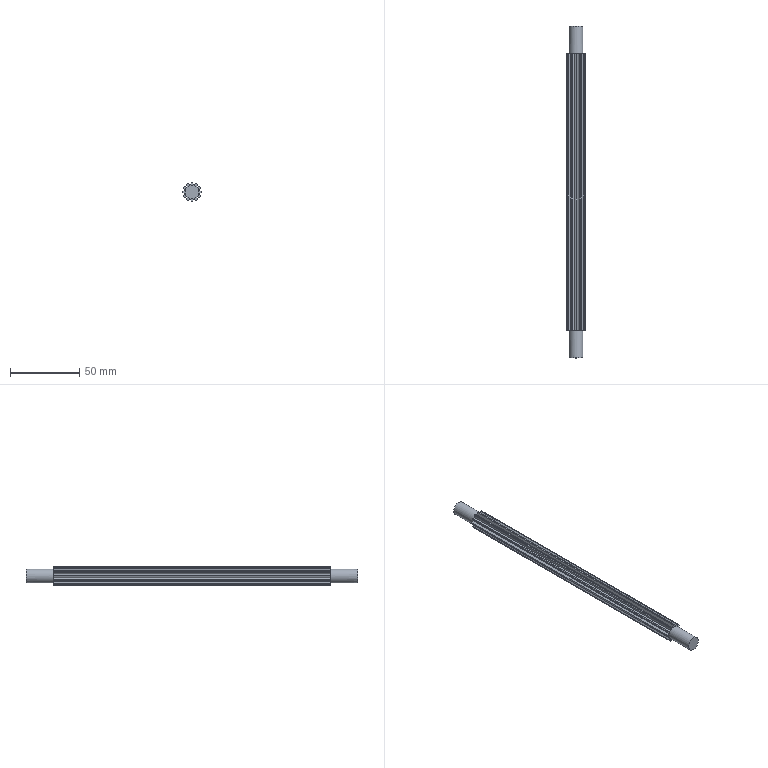Component | NX | MODEL5 | 1 solid | 75 faces | volume 26630 mm3 | plane 74 | cylinder 1 | commonest cylinder face diameters 10 x1